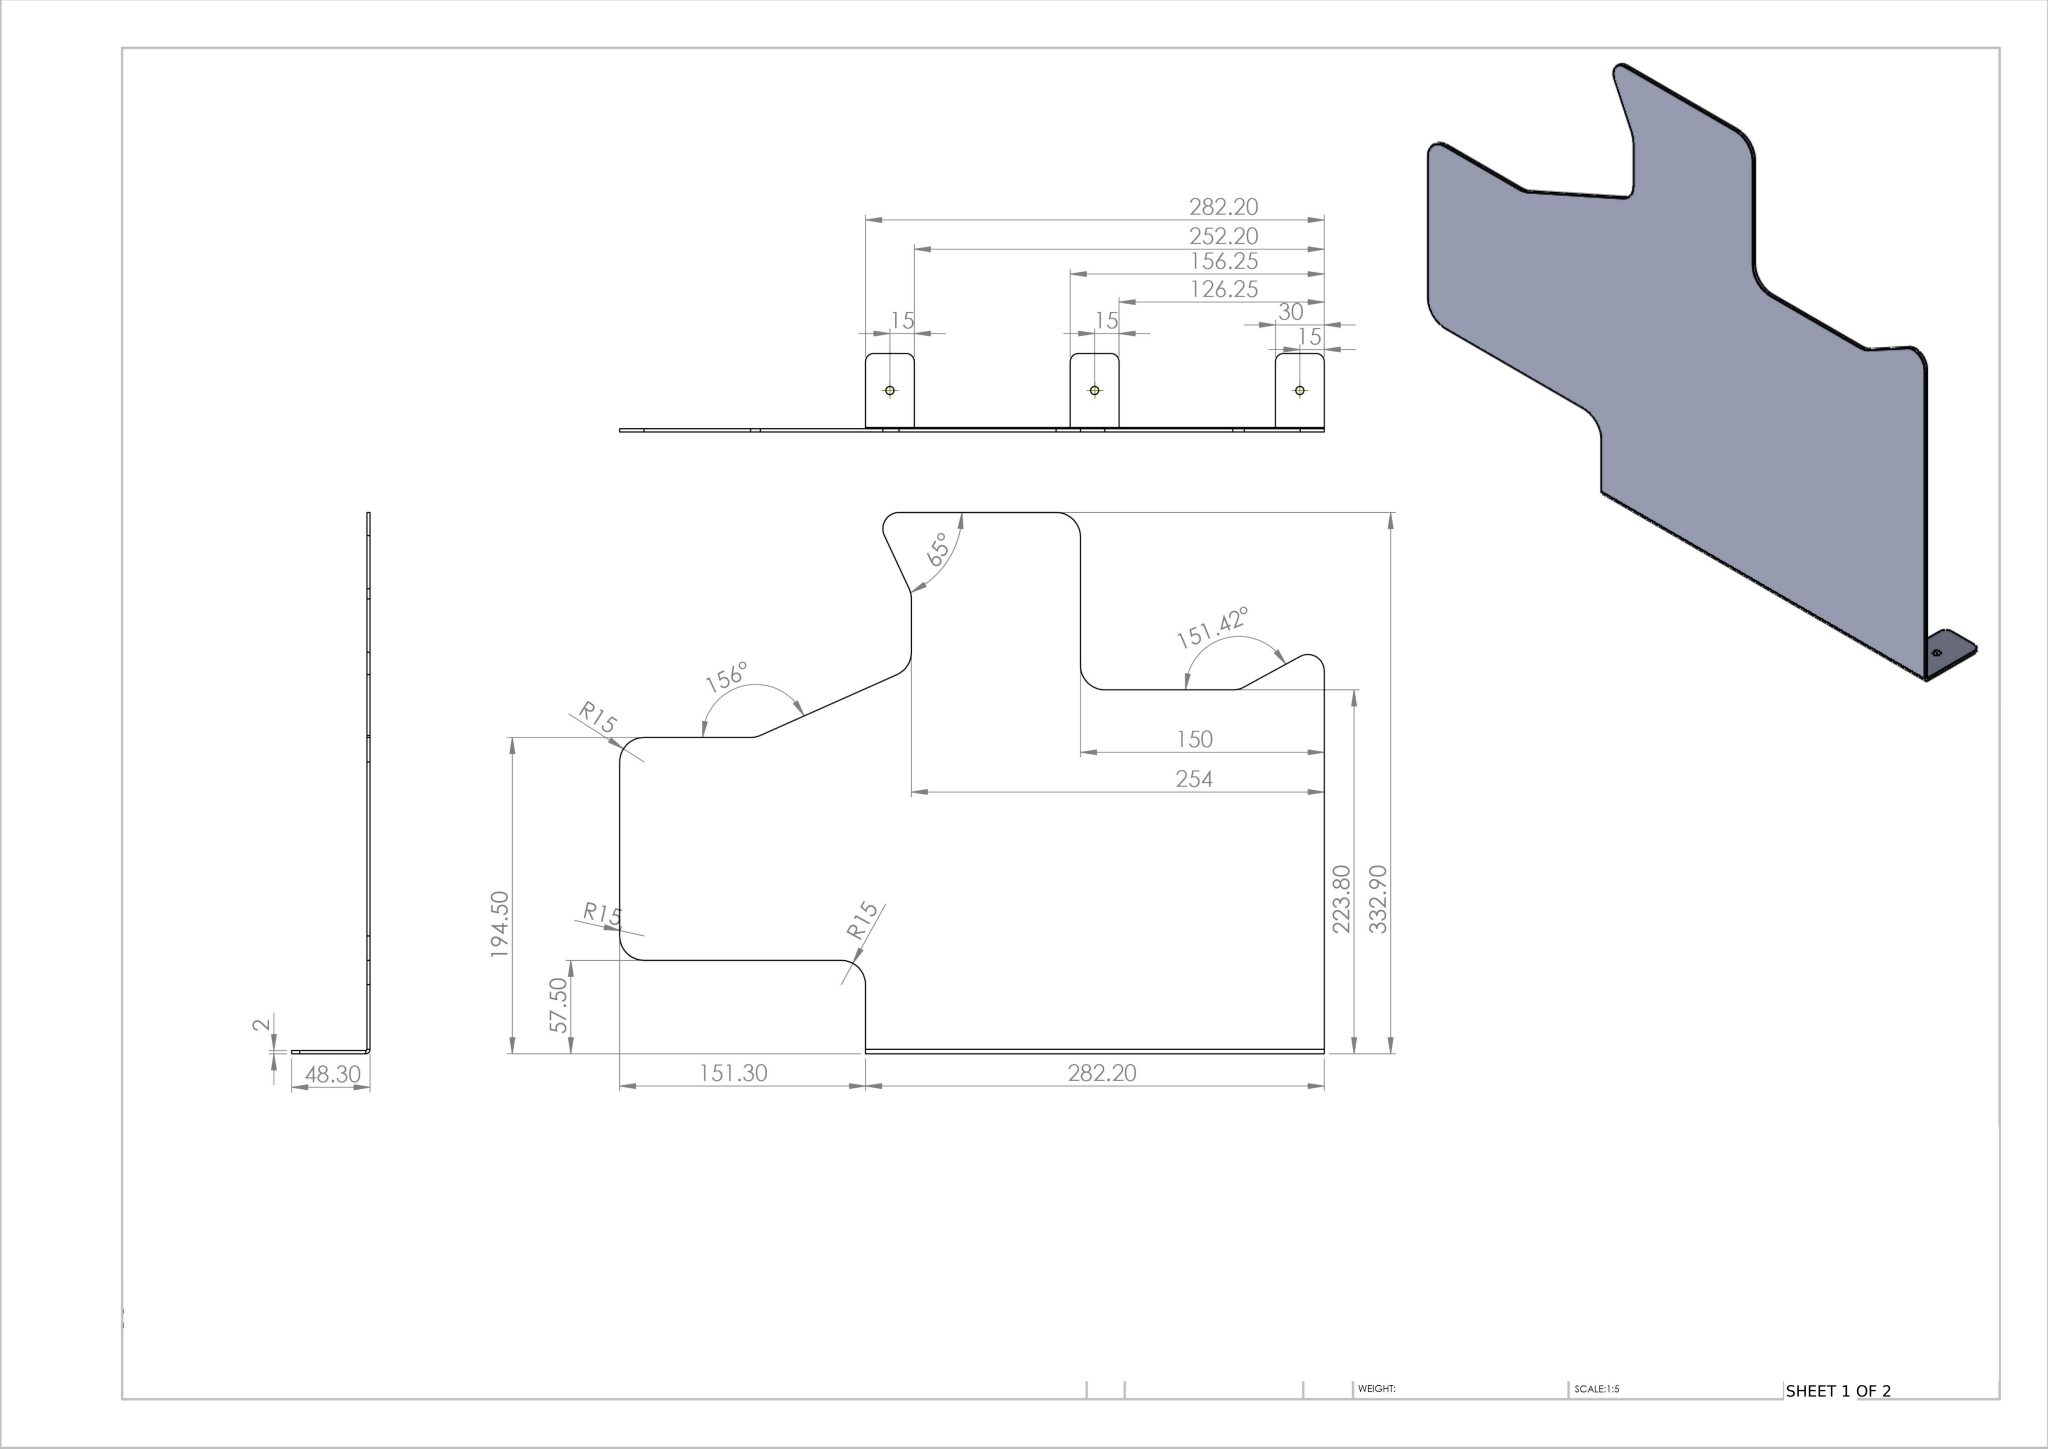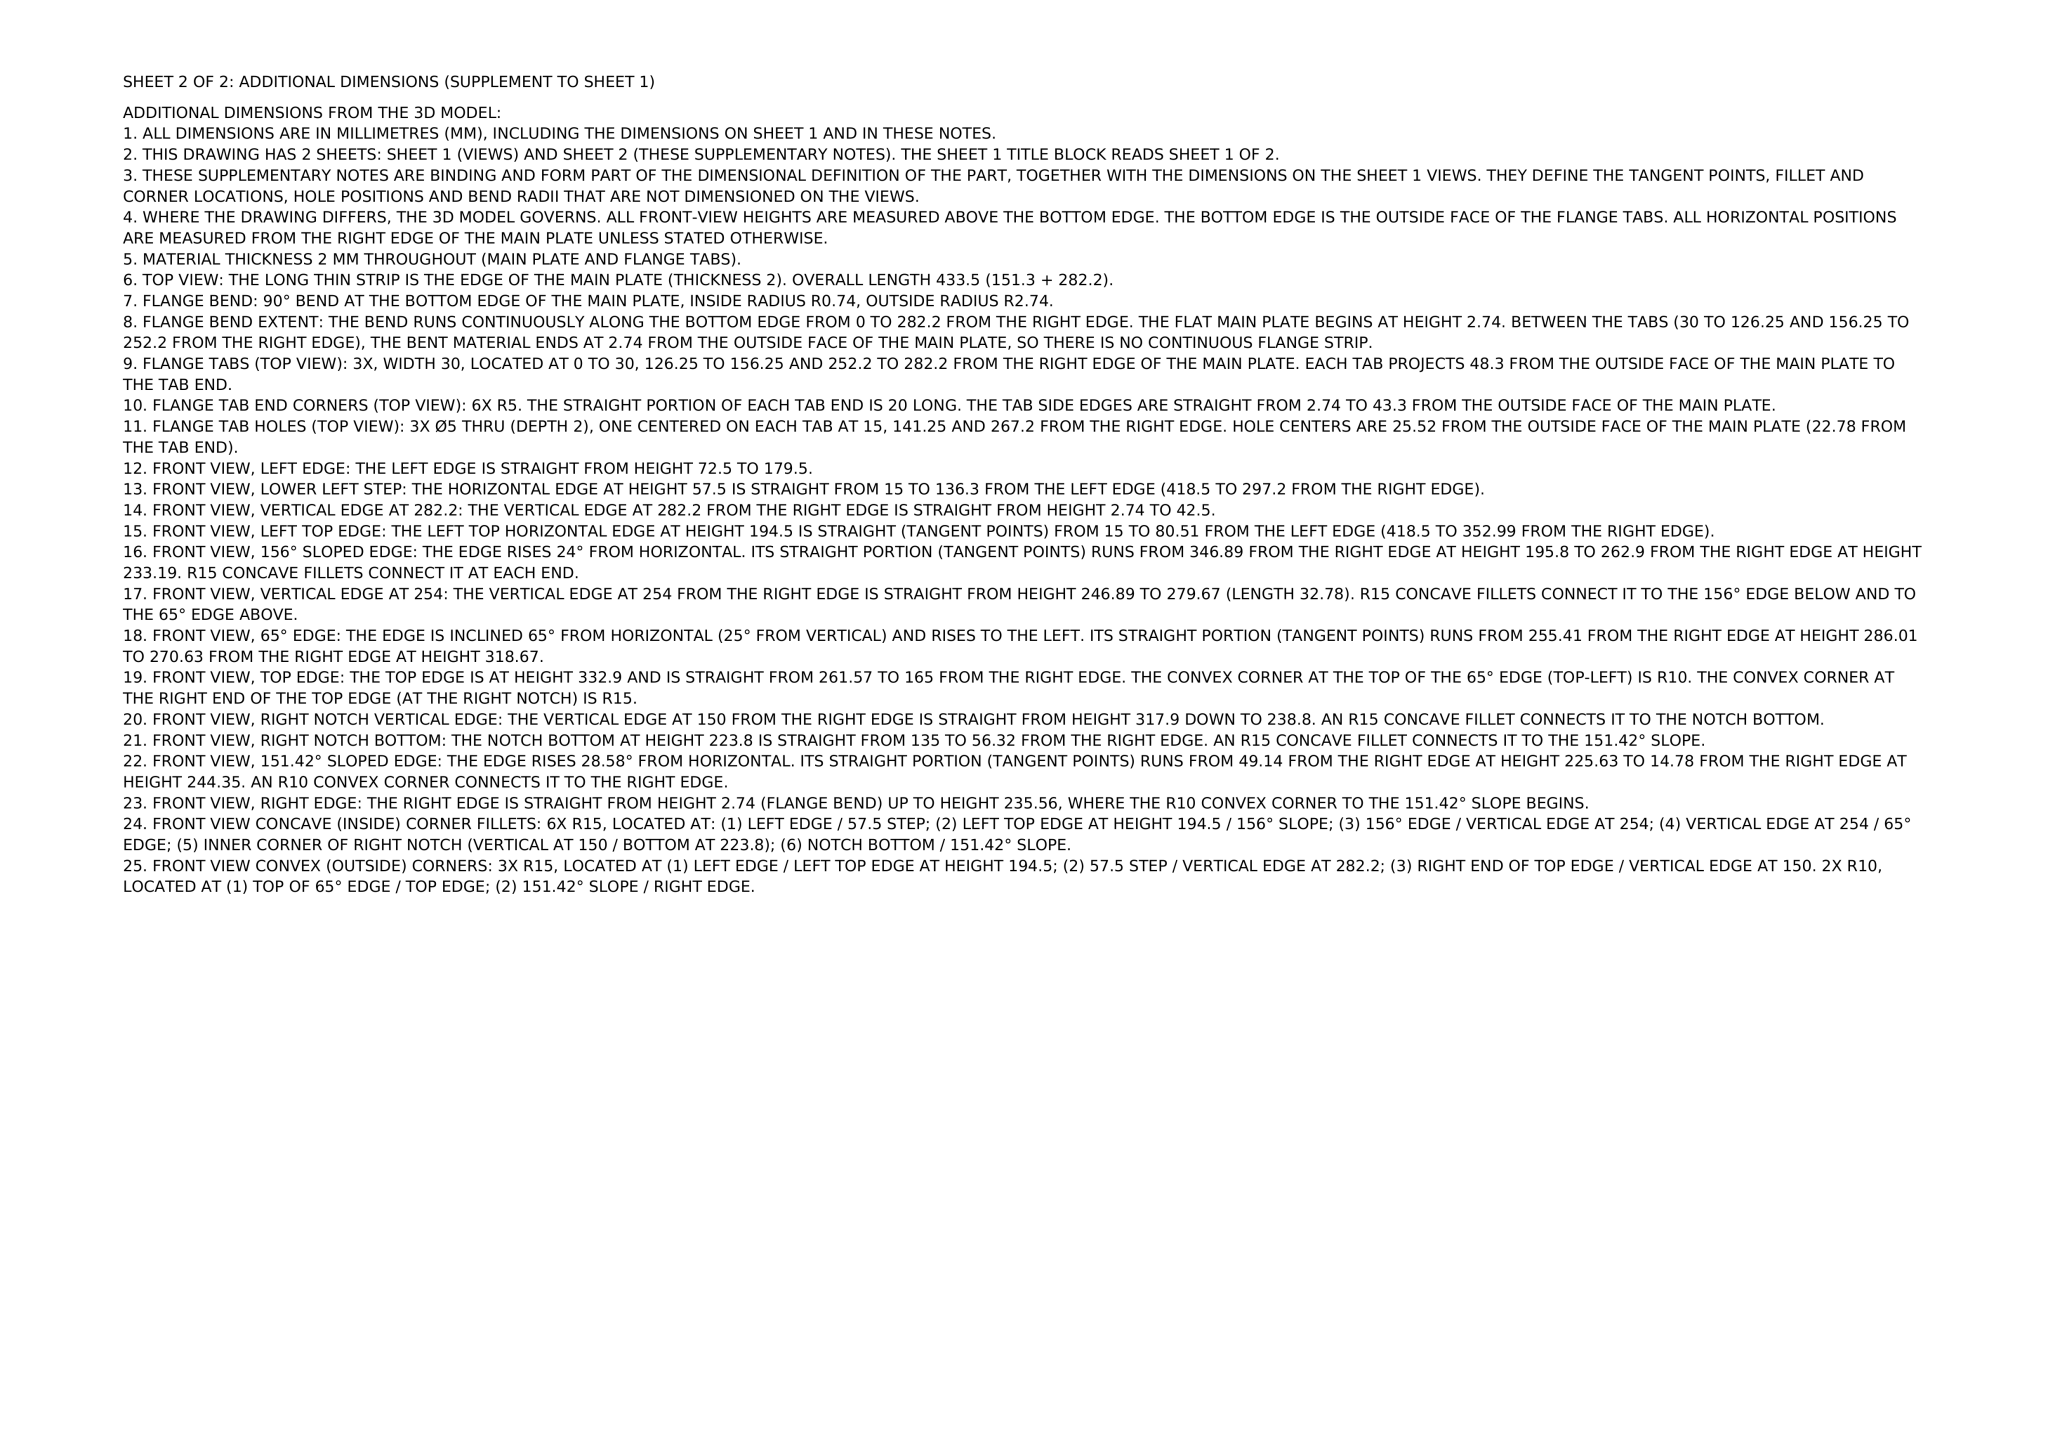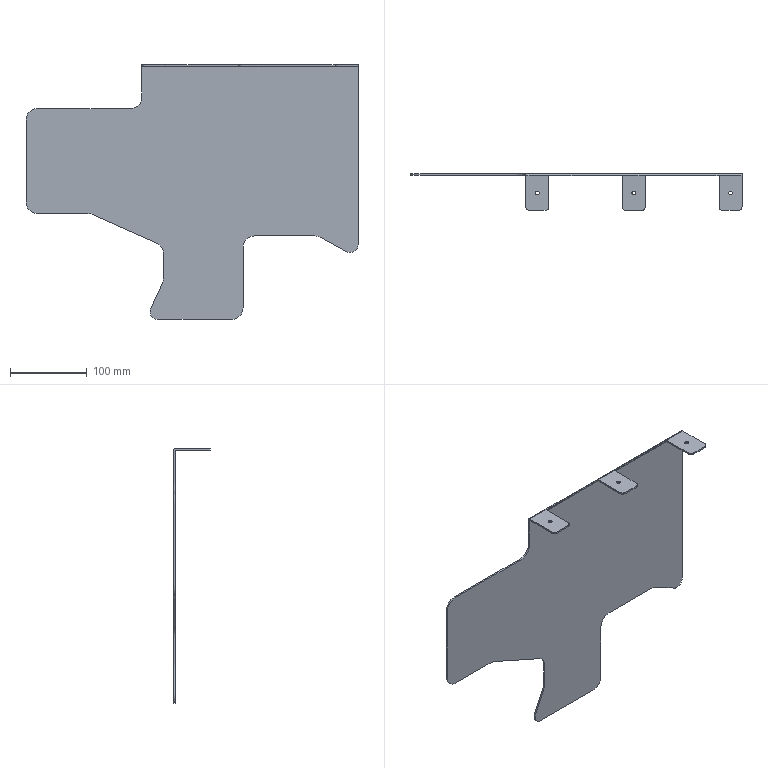Part | NX | mm | 1 solid | 59 faces | box 433.5 x 48.3 x 332.9 mm | volume 203271 mm3 | plane 33 | cylinder 26 | commonest cylinder face diameters 30 x9 5 x6 10 x6 20 x3 1.473 x1 5.473 x1